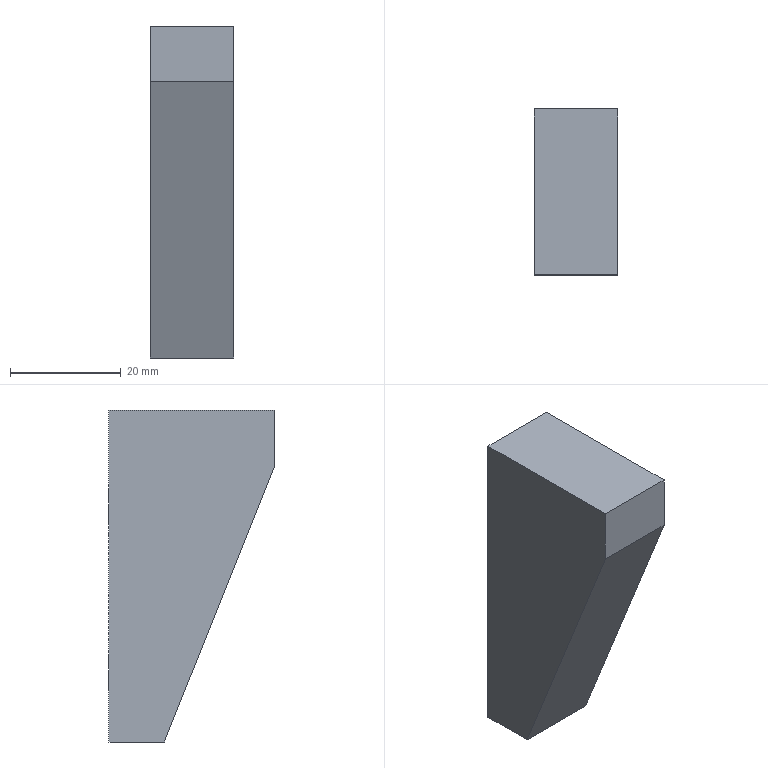Component | NX | REINFORCE_RIB_2 | 1 solid | 13 faces | box 15 x 30 x 60 mm | volume 18782 mm3 | plane 7 | cone 4 | cylinder 2 | commonest cylinder face diameters 6 x2
STEP:
#1=CARTESIAN_POINT('',(0.,0.,0.));
#2=DIRECTION('',(0.,0.,1.));
#3=DIRECTION('',(1.,0.,0.));
#4=AXIS2_PLACEMENT_3D('',#1,#2,#3);
#5=CARTESIAN_POINT('',(-1.906,179.462,226.966));
#6=VERTEX_POINT('',#5);
#7=CARTESIAN_POINT('',(-1.906,179.462,223.466));
#8=DIRECTION('',(0.,-1.,0.));
#9=DIRECTION('',(0.,0.,1.));
#10=AXIS2_PLACEMENT_3D('',#7,#8,#9);
#11=CIRCLE('',#10,3.5);
#12=CARTESIAN_POINT('',(-9.406,179.462,270.466));
#13=DIRECTION('',(0.,-1.,0.));
#14=DIRECTION('',(0.,0.,1.));
#15=AXIS2_PLACEMENT_3D('',#12,#13,#14);
#16=PLANE('',#15);
#17=CARTESIAN_POINT('',(-47.,-7.5));
#18=DIRECTION('',(1.,0.));
#19=AXIS2_PLACEMENT_2D('',#17,#18);
#20=CIRCLE('',#19,3.5);
#21=(GEOMETRIC_REPRESENTATION_CONTEXT(2)PARAMETRIC_REPRESENTATION_CONTEXT()REPRESENTATION_CONTEXT('',''));
#22=DEFINITIONAL_REPRESENTATION('',(#20),#21);
#23=PCURVE('',#16,#22);
#24=CARTESIAN_POINT('',(-1.906,179.462,223.466));
#25=DIRECTION('',(0.,1.,0.));
#26=DIRECTION('',(-1.,0.,0.));
#27=AXIS2_PLACEMENT_3D('',#24,#25,#26);
#28=CONICAL_SURFACE('',#27,3.5,0.7854);
#29=CARTESIAN_POINT('',(7.854,0.));
#30=DIRECTION('',(-1.,0.));
#31=VECTOR('',#30,1.);
#32=LINE('',#29,#31);
#33=(GEOMETRIC_REPRESENTATION_CONTEXT(2)PARAMETRIC_REPRESENTATION_CONTEXT()REPRESENTATION_CONTEXT('',''));
#34=DEFINITIONAL_REPRESENTATION('',(#32),#33);
#35=PCURVE('',#28,#34);
#36=SURFACE_CURVE('',#11,(#23,#35),.PCURVE_S1.);
#37=EDGE_CURVE('',#6,#6,#36,.T.);
#38=ORIENTED_EDGE('',*,*,#37,.T.);
#39=EDGE_LOOP('',(#38));
#40=FACE_BOUND('',#39,.T.);
#41=CARTESIAN_POINT('',(-1.906,179.462,256.966));
#42=VERTEX_POINT('',#41);
#43=CARTESIAN_POINT('',(-1.906,179.462,253.466));
#44=DIRECTION('',(0.,-1.,0.));
#45=DIRECTION('',(0.,0.,1.));
#46=AXIS2_PLACEMENT_3D('',#43,#44,#45);
#47=CIRCLE('',#46,3.5);
#48=CARTESIAN_POINT('',(-17.,-7.5));
#49=DIRECTION('',(1.,0.));
#50=AXIS2_PLACEMENT_2D('',#48,#49);
#51=CIRCLE('',#50,3.5);
#52=(GEOMETRIC_REPRESENTATION_CONTEXT(2)PARAMETRIC_REPRESENTATION_CONTEXT()REPRESENTATION_CONTEXT('',''));
#53=DEFINITIONAL_REPRESENTATION('',(#51),#52);
#54=PCURVE('',#16,#53);
#55=CARTESIAN_POINT('',(-1.906,179.462,253.466));
#56=DIRECTION('',(0.,1.,0.));
#57=DIRECTION('',(-1.,0.,0.));
#58=AXIS2_PLACEMENT_3D('',#55,#56,#57);
#59=CONICAL_SURFACE('',#58,3.5,0.7854);
#60=CARTESIAN_POINT('',(7.854,0.));
#61=DIRECTION('',(-1.,0.));
#62=VECTOR('',#61,1.);
#63=LINE('',#60,#62);
#64=(GEOMETRIC_REPRESENTATION_CONTEXT(2)PARAMETRIC_REPRESENTATION_CONTEXT()REPRESENTATION_CONTEXT('',''));
#65=DEFINITIONAL_REPRESENTATION('',(#63),#64);
#66=PCURVE('',#59,#65);
#67=SURFACE_CURVE('',#47,(#54,#66),.PCURVE_S1.);
#68=EDGE_CURVE('',#42,#42,#67,.T.);
#69=ORIENTED_EDGE('',*,*,#68,.T.);
#70=EDGE_LOOP('',(#69));
#71=FACE_BOUND('',#70,.T.);
#72=CARTESIAN_POINT('',(5.594,179.462,270.466));
#73=VERTEX_POINT('',#72);
#74=CARTESIAN_POINT('',(5.594,179.462,210.466));
#75=VERTEX_POINT('',#74);
#76=CARTESIAN_POINT('',(5.594,179.462,270.466));
#77=DIRECTION('',(0.,-0.,-1.));
#78=VECTOR('',#77,1.);
#79=LINE('',#76,#78);
#80=CARTESIAN_POINT('',(0.,-15.));
#81=DIRECTION('',(-1.,0.));
#82=VECTOR('',#81,1.);
#83=LINE('',#80,#82);
#84=(GEOMETRIC_REPRESENTATION_CONTEXT(2)PARAMETRIC_REPRESENTATION_CONTEXT()REPRESENTATION_CONTEXT('',''));
#85=DEFINITIONAL_REPRESENTATION('',(#83),#84);
#86=PCURVE('',#16,#85);
#87=CARTESIAN_POINT('',(5.594,179.462,210.466));
#88=DIRECTION('',(-1.,0.,0.));
#89=DIRECTION('',(0.,-1.,0.));
#90=AXIS2_PLACEMENT_3D('',#87,#88,#89);
#91=PLANE('',#90);
#92=CARTESIAN_POINT('',(0.,60.));
#93=DIRECTION('',(0.,-1.));
#94=VECTOR('',#93,1.);
#95=LINE('',#92,#94);
#96=(GEOMETRIC_REPRESENTATION_CONTEXT(2)PARAMETRIC_REPRESENTATION_CONTEXT()REPRESENTATION_CONTEXT('',''));
#97=DEFINITIONAL_REPRESENTATION('',(#95),#96);
#98=PCURVE('',#91,#97);
#99=SURFACE_CURVE('',#79,(#86,#98),.PCURVE_S1.);
#100=EDGE_CURVE('',#73,#75,#99,.T.);
#101=ORIENTED_EDGE('',*,*,#100,.T.);
#102=CARTESIAN_POINT('',(-9.406,179.462,210.466));
#103=VERTEX_POINT('',#102);
#104=CARTESIAN_POINT('',(-9.406,179.462,210.466));
#105=DIRECTION('',(1.,0.,0.));
#106=VECTOR('',#105,1.);
#107=LINE('',#104,#106);
#108=CARTESIAN_POINT('',(-60.,0.));
#109=DIRECTION('',(0.,-1.));
#110=VECTOR('',#109,1.);
#111=LINE('',#108,#110);
#112=(GEOMETRIC_REPRESENTATION_CONTEXT(2)PARAMETRIC_REPRESENTATION_CONTEXT()REPRESENTATION_CONTEXT('',''));
#113=DEFINITIONAL_REPRESENTATION('',(#111),#112);
#114=PCURVE('',#16,#113);
#115=CARTESIAN_POINT('',(-9.406,179.462,210.466));
#116=DIRECTION('',(0.,0.,1.));
#117=DIRECTION('',(-1.,0.,0.));
#118=AXIS2_PLACEMENT_3D('',#115,#116,#117);
#119=PLANE('',#118);
#120=CARTESIAN_POINT('',(0.,0.));
#121=DIRECTION('',(-1.,0.));
#122=VECTOR('',#121,1.);
#123=LINE('',#120,#122);
#124=(GEOMETRIC_REPRESENTATION_CONTEXT(2)PARAMETRIC_REPRESENTATION_CONTEXT()REPRESENTATION_CONTEXT('',''));
#125=DEFINITIONAL_REPRESENTATION('',(#123),#124);
#126=PCURVE('',#119,#125);
#127=SURFACE_CURVE('',#107,(#114,#126),.PCURVE_S1.);
#128=EDGE_CURVE('',#103,#75,#127,.T.);
#129=ORIENTED_EDGE('',*,*,#128,.F.);
#130=CARTESIAN_POINT('',(-9.406,179.462,270.466));
#131=VERTEX_POINT('',#130);
#132=CARTESIAN_POINT('',(-9.406,179.462,270.466));
#133=DIRECTION('',(0.,-0.,-1.));
#134=VECTOR('',#133,1.);
#135=LINE('',#132,#134);
#136=CARTESIAN_POINT('',(0.,0.));
#137=DIRECTION('',(-1.,0.));
#138=VECTOR('',#137,1.);
#139=LINE('',#136,#138);
#140=(GEOMETRIC_REPRESENTATION_CONTEXT(2)PARAMETRIC_REPRESENTATION_CONTEXT()REPRESENTATION_CONTEXT('',''));
#141=DEFINITIONAL_REPRESENTATION('',(#139),#140);
#142=PCURVE('',#16,#141);
#143=CARTESIAN_POINT('',(-9.406,179.462,210.466));
#144=DIRECTION('',(-1.,0.,0.));
#145=DIRECTION('',(0.,-1.,0.));
#146=AXIS2_PLACEMENT_3D('',#143,#144,#145);
#147=PLANE('',#146);
#148=CARTESIAN_POINT('',(0.,60.));
#149=DIRECTION('',(0.,-1.));
#150=VECTOR('',#149,1.);
#151=LINE('',#148,#150);
#152=(GEOMETRIC_REPRESENTATION_CONTEXT(2)PARAMETRIC_REPRESENTATION_CONTEXT()REPRESENTATION_CONTEXT('',''));
#153=DEFINITIONAL_REPRESENTATION('',(#151),#152);
#154=PCURVE('',#147,#153);
#155=SURFACE_CURVE('',#135,(#142,#154),.PCURVE_S1.);
#156=EDGE_CURVE('',#131,#103,#155,.T.);
#157=ORIENTED_EDGE('',*,*,#156,.F.);
#158=CARTESIAN_POINT('',(-9.406,179.462,270.466));
#159=DIRECTION('',(1.,0.,0.));
#160=VECTOR('',#159,1.);
#161=LINE('',#158,#160);
#162=CARTESIAN_POINT('',(0.,0.));
#163=DIRECTION('',(0.,-1.));
#164=VECTOR('',#163,1.);
#165=LINE('',#162,#164);
#166=(GEOMETRIC_REPRESENTATION_CONTEXT(2)PARAMETRIC_REPRESENTATION_CONTEXT()REPRESENTATION_CONTEXT('',''));
#167=DEFINITIONAL_REPRESENTATION('',(#165),#166);
#168=PCURVE('',#16,#167);
#169=CARTESIAN_POINT('',(-9.406,149.462,270.466));
#170=DIRECTION('',(0.,0.,-1.));
#171=DIRECTION('',(1.,0.,0.));
#172=AXIS2_PLACEMENT_3D('',#169,#170,#171);
#173=PLANE('',#172);
#174=CARTESIAN_POINT('',(0.,-30.));
#175=DIRECTION('',(1.,0.));
#176=VECTOR('',#175,1.);
#177=LINE('',#174,#176);
#178=(GEOMETRIC_REPRESENTATION_CONTEXT(2)PARAMETRIC_REPRESENTATION_CONTEXT()REPRESENTATION_CONTEXT('',''));
#179=DEFINITIONAL_REPRESENTATION('',(#177),#178);
#180=PCURVE('',#173,#179);
#181=SURFACE_CURVE('',#161,(#168,#180),.PCURVE_S1.);
#182=EDGE_CURVE('',#131,#73,#181,.T.);
#183=ORIENTED_EDGE('',*,*,#182,.T.);
#184=EDGE_LOOP('',(#101,#129,#157,#183));
#185=FACE_BOUND('',#184,.T.);
#186=ADVANCED_FACE('',(#40,#71,#185),#16,.F.);
#187=CARTESIAN_POINT('',(5.594,169.462,210.466));
#188=VERTEX_POINT('',#187);
#189=CARTESIAN_POINT('',(5.594,179.462,210.466));
#190=DIRECTION('',(0.,-1.,0.));
#191=VECTOR('',#190,1.);
#192=LINE('',#189,#191);
#193=CARTESIAN_POINT('',(-15.,0.));
#194=DIRECTION('',(0.,1.));
#195=VECTOR('',#194,1.);
#196=LINE('',#193,#195);
#197=(GEOMETRIC_REPRESENTATION_CONTEXT(2)PARAMETRIC_REPRESENTATION_CONTEXT()REPRESENTATION_CONTEXT('',''));
#198=DEFINITIONAL_REPRESENTATION('',(#196),#197);
#199=PCURVE('',#119,#198);
#200=CARTESIAN_POINT('',(0.,0.));
#201=DIRECTION('',(1.,0.));
#202=VECTOR('',#201,1.);
#203=LINE('',#200,#202);
#204=(GEOMETRIC_REPRESENTATION_CONTEXT(2)PARAMETRIC_REPRESENTATION_CONTEXT()REPRESENTATION_CONTEXT('',''));
#205=DEFINITIONAL_REPRESENTATION('',(#203),#204);
#206=PCURVE('',#91,#205);
#207=SURFACE_CURVE('',#192,(#199,#206),.PCURVE_S1.);
#208=EDGE_CURVE('',#75,#188,#207,.T.);
#209=ORIENTED_EDGE('',*,*,#208,.T.);
#210=CARTESIAN_POINT('',(-9.406,169.462,210.466));
#211=VERTEX_POINT('',#210);
#212=CARTESIAN_POINT('',(-9.406,169.462,210.466));
#213=DIRECTION('',(1.,0.,0.));
#214=VECTOR('',#213,1.);
#215=LINE('',#212,#214);
#216=CARTESIAN_POINT('',(0.,10.));
#217=DIRECTION('',(-1.,0.));
#218=VECTOR('',#217,1.);
#219=LINE('',#216,#218);
#220=(GEOMETRIC_REPRESENTATION_CONTEXT(2)PARAMETRIC_REPRESENTATION_CONTEXT()REPRESENTATION_CONTEXT('',''));
#221=DEFINITIONAL_REPRESENTATION('',(#219),#220);
#222=PCURVE('',#119,#221);
#223=CARTESIAN_POINT('',(-9.406,169.462,210.466));
#224=DIRECTION('',(0.,0.9285,0.3714));
#225=DIRECTION('',(0.,0.3714,-0.9285));
#226=AXIS2_PLACEMENT_3D('',#223,#224,#225);
#227=PLANE('',#226);
#228=CARTESIAN_POINT('',(0.,0.));
#229=DIRECTION('',(0.,-1.));
#230=VECTOR('',#229,1.);
#231=LINE('',#228,#230);
#232=(GEOMETRIC_REPRESENTATION_CONTEXT(2)PARAMETRIC_REPRESENTATION_CONTEXT()REPRESENTATION_CONTEXT('',''));
#233=DEFINITIONAL_REPRESENTATION('',(#231),#232);
#234=PCURVE('',#227,#233);
#235=SURFACE_CURVE('',#215,(#222,#234),.PCURVE_S1.);
#236=EDGE_CURVE('',#211,#188,#235,.T.);
#237=ORIENTED_EDGE('',*,*,#236,.F.);
#238=CARTESIAN_POINT('',(-9.406,179.462,210.466));
#239=DIRECTION('',(0.,-1.,0.));
#240=VECTOR('',#239,1.);
#241=LINE('',#238,#240);
#242=CARTESIAN_POINT('',(0.,0.));
#243=DIRECTION('',(0.,1.));
#244=VECTOR('',#243,1.);
#245=LINE('',#242,#244);
#246=(GEOMETRIC_REPRESENTATION_CONTEXT(2)PARAMETRIC_REPRESENTATION_CONTEXT()REPRESENTATION_CONTEXT('',''));
#247=DEFINITIONAL_REPRESENTATION('',(#245),#246);
#248=PCURVE('',#119,#247);
#249=CARTESIAN_POINT('',(0.,0.));
#250=DIRECTION('',(1.,0.));
#251=VECTOR('',#250,1.);
#252=LINE('',#249,#251);
#253=(GEOMETRIC_REPRESENTATION_CONTEXT(2)PARAMETRIC_REPRESENTATION_CONTEXT()REPRESENTATION_CONTEXT('',''));
#254=DEFINITIONAL_REPRESENTATION('',(#252),#253);
#255=PCURVE('',#147,#254);
#256=SURFACE_CURVE('',#241,(#248,#255),.PCURVE_S1.);
#257=EDGE_CURVE('',#103,#211,#256,.T.);
#258=ORIENTED_EDGE('',*,*,#257,.F.);
#259=ORIENTED_EDGE('',*,*,#128,.T.);
#260=EDGE_LOOP('',(#209,#237,#258,#259));
#261=FACE_BOUND('',#260,.T.);
#262=ADVANCED_FACE('',(#261),#119,.F.);
#263=CARTESIAN_POINT('',(5.594,149.462,260.466));
#264=VERTEX_POINT('',#263);
#265=CARTESIAN_POINT('',(5.594,169.462,210.466));
#266=DIRECTION('',(0.,-0.3714,0.9285));
#267=VECTOR('',#266,1.);
#268=LINE('',#265,#267);
#269=CARTESIAN_POINT('',(0.,-15.));
#270=DIRECTION('',(-1.,0.));
#271=VECTOR('',#270,1.);
#272=LINE('',#269,#271);
#273=(GEOMETRIC_REPRESENTATION_CONTEXT(2)PARAMETRIC_REPRESENTATION_CONTEXT()REPRESENTATION_CONTEXT('',''));
#274=DEFINITIONAL_REPRESENTATION('',(#272),#273);
#275=PCURVE('',#227,#274);
#276=CARTESIAN_POINT('',(10.,0.));
#277=DIRECTION('',(0.3714,0.9285));
#278=VECTOR('',#277,1.);
#279=LINE('',#276,#278);
#280=(GEOMETRIC_REPRESENTATION_CONTEXT(2)PARAMETRIC_REPRESENTATION_CONTEXT()REPRESENTATION_CONTEXT('',''));
#281=DEFINITIONAL_REPRESENTATION('',(#279),#280);
#282=PCURVE('',#91,#281);
#283=SURFACE_CURVE('',#268,(#275,#282),.PCURVE_S1.);
#284=EDGE_CURVE('',#188,#264,#283,.T.);
#285=ORIENTED_EDGE('',*,*,#284,.T.);
#286=CARTESIAN_POINT('',(-9.406,149.462,260.466));
#287=VERTEX_POINT('',#286);
#288=CARTESIAN_POINT('',(-9.406,149.462,260.466));
#289=DIRECTION('',(1.,0.,0.));
#290=VECTOR('',#289,1.);
#291=LINE('',#288,#290);
#292=CARTESIAN_POINT('',(-53.852,0.));
#293=DIRECTION('',(0.,-1.));
#294=VECTOR('',#293,1.);
#295=LINE('',#292,#294);
#296=(GEOMETRIC_REPRESENTATION_CONTEXT(2)PARAMETRIC_REPRESENTATION_CONTEXT()REPRESENTATION_CONTEXT('',''));
#297=DEFINITIONAL_REPRESENTATION('',(#295),#296);
#298=PCURVE('',#227,#297);
#299=CARTESIAN_POINT('',(-9.406,149.462,260.466));
#300=DIRECTION('',(0.,1.,0.));
#301=DIRECTION('',(-1.,0.,0.));
#302=AXIS2_PLACEMENT_3D('',#299,#300,#301);
#303=PLANE('',#302);
#304=CARTESIAN_POINT('',(0.,0.));
#305=DIRECTION('',(-1.,0.));
#306=VECTOR('',#305,1.);
#307=LINE('',#304,#306);
#308=(GEOMETRIC_REPRESENTATION_CONTEXT(2)PARAMETRIC_REPRESENTATION_CONTEXT()REPRESENTATION_CONTEXT('',''));
#309=DEFINITIONAL_REPRESENTATION('',(#307),#308);
#310=PCURVE('',#303,#309);
#311=SURFACE_CURVE('',#291,(#298,#310),.PCURVE_S1.);
#312=EDGE_CURVE('',#287,#264,#311,.T.);
#313=ORIENTED_EDGE('',*,*,#312,.F.);
#314=CARTESIAN_POINT('',(-9.406,169.462,210.466));
#315=DIRECTION('',(0.,-0.3714,0.9285));
#316=VECTOR('',#315,1.);
#317=LINE('',#314,#316);
#318=CARTESIAN_POINT('',(0.,0.));
#319=DIRECTION('',(-1.,0.));
#320=VECTOR('',#319,1.);
#321=LINE('',#318,#320);
#322=(GEOMETRIC_REPRESENTATION_CONTEXT(2)PARAMETRIC_REPRESENTATION_CONTEXT()REPRESENTATION_CONTEXT('',''));
#323=DEFINITIONAL_REPRESENTATION('',(#321),#322);
#324=PCURVE('',#227,#323);
#325=CARTESIAN_POINT('',(10.,0.));
#326=DIRECTION('',(0.3714,0.9285));
#327=VECTOR('',#326,1.);
#328=LINE('',#325,#327);
#329=(GEOMETRIC_REPRESENTATION_CONTEXT(2)PARAMETRIC_REPRESENTATION_CONTEXT()REPRESENTATION_CONTEXT('',''));
#330=DEFINITIONAL_REPRESENTATION('',(#328),#329);
#331=PCURVE('',#147,#330);
#332=SURFACE_CURVE('',#317,(#324,#331),.PCURVE_S1.);
#333=EDGE_CURVE('',#211,#287,#332,.T.);
#334=ORIENTED_EDGE('',*,*,#333,.F.);
#335=ORIENTED_EDGE('',*,*,#236,.T.);
#336=EDGE_LOOP('',(#285,#313,#334,#335));
#337=FACE_BOUND('',#336,.T.);
#338=ADVANCED_FACE('',(#337),#227,.F.);
#339=CARTESIAN_POINT('',(5.594,149.462,270.466));
#340=VERTEX_POINT('',#339);
#341=CARTESIAN_POINT('',(5.594,149.462,260.466));
#342=DIRECTION('',(0.,0.,1.));
#343=VECTOR('',#342,1.);
#344=LINE('',#341,#343);
#345=CARTESIAN_POINT('',(-15.,0.));
#346=DIRECTION('',(0.,1.));
#347=VECTOR('',#346,1.);
#348=LINE('',#345,#347);
#349=(GEOMETRIC_REPRESENTATION_CONTEXT(2)PARAMETRIC_REPRESENTATION_CONTEXT()REPRESENTATION_CONTEXT('',''));
#350=DEFINITIONAL_REPRESENTATION('',(#348),#349);
#351=PCURVE('',#303,#350);
#352=CARTESIAN_POINT('',(30.,50.));
#353=DIRECTION('',(0.,1.));
#354=VECTOR('',#353,1.);
#355=LINE('',#352,#354);
#356=(GEOMETRIC_REPRESENTATION_CONTEXT(2)PARAMETRIC_REPRESENTATION_CONTEXT()REPRESENTATION_CONTEXT('',''));
#357=DEFINITIONAL_REPRESENTATION('',(#355),#356);
#358=PCURVE('',#91,#357);
#359=SURFACE_CURVE('',#344,(#351,#358),.PCURVE_S1.);
#360=EDGE_CURVE('',#264,#340,#359,.T.);
#361=ORIENTED_EDGE('',*,*,#360,.T.);
#362=CARTESIAN_POINT('',(-9.406,149.462,270.466));
#363=VERTEX_POINT('',#362);
#364=CARTESIAN_POINT('',(-9.406,149.462,270.466));
#365=DIRECTION('',(1.,0.,0.));
#366=VECTOR('',#365,1.);
#367=LINE('',#364,#366);
#368=CARTESIAN_POINT('',(0.,10.));
#369=DIRECTION('',(-1.,0.));
#370=VECTOR('',#369,1.);
#371=LINE('',#368,#370);
#372=(GEOMETRIC_REPRESENTATION_CONTEXT(2)PARAMETRIC_REPRESENTATION_CONTEXT()REPRESENTATION_CONTEXT('',''));
#373=DEFINITIONAL_REPRESENTATION('',(#371),#372);
#374=PCURVE('',#303,#373);
#375=CARTESIAN_POINT('',(0.,0.));
#376=DIRECTION('',(1.,0.));
#377=VECTOR('',#376,1.);
#378=LINE('',#375,#377);
#379=(GEOMETRIC_REPRESENTATION_CONTEXT(2)PARAMETRIC_REPRESENTATION_CONTEXT()REPRESENTATION_CONTEXT('',''));
#380=DEFINITIONAL_REPRESENTATION('',(#378),#379);
#381=PCURVE('',#173,#380);
#382=SURFACE_CURVE('',#367,(#374,#381),.PCURVE_S1.);
#383=EDGE_CURVE('',#363,#340,#382,.T.);
#384=ORIENTED_EDGE('',*,*,#383,.F.);
#385=CARTESIAN_POINT('',(-9.406,149.462,260.466));
#386=DIRECTION('',(0.,0.,1.));
#387=VECTOR('',#386,1.);
#388=LINE('',#385,#387);
#389=CARTESIAN_POINT('',(0.,0.));
#390=DIRECTION('',(0.,1.));
#391=VECTOR('',#390,1.);
#392=LINE('',#389,#391);
#393=(GEOMETRIC_REPRESENTATION_CONTEXT(2)PARAMETRIC_REPRESENTATION_CONTEXT()REPRESENTATION_CONTEXT('',''));
#394=DEFINITIONAL_REPRESENTATION('',(#392),#393);
#395=PCURVE('',#303,#394);
#396=CARTESIAN_POINT('',(30.,50.));
#397=DIRECTION('',(0.,1.));
#398=VECTOR('',#397,1.);
#399=LINE('',#396,#398);
#400=(GEOMETRIC_REPRESENTATION_CONTEXT(2)PARAMETRIC_REPRESENTATION_CONTEXT()REPRESENTATION_CONTEXT('',''));
#401=DEFINITIONAL_REPRESENTATION('',(#399),#400);
#402=PCURVE('',#147,#401);
#403=SURFACE_CURVE('',#388,(#395,#402),.PCURVE_S1.);
#404=EDGE_CURVE('',#287,#363,#403,.T.);
#405=ORIENTED_EDGE('',*,*,#404,.F.);
#406=ORIENTED_EDGE('',*,*,#312,.T.);
#407=EDGE_LOOP('',(#361,#384,#405,#406));
#408=FACE_BOUND('',#407,.T.);
#409=ADVANCED_FACE('',(#408),#303,.F.);
#410=CARTESIAN_POINT('',(5.594,149.462,270.466));
#411=DIRECTION('',(0.,1.,0.));
#412=VECTOR('',#411,1.);
#413=LINE('',#410,#412);
#414=CARTESIAN_POINT('',(15.,0.));
#415=DIRECTION('',(0.,-1.));
#416=VECTOR('',#415,1.);
#417=LINE('',#414,#416);
#418=(GEOMETRIC_REPRESENTATION_CONTEXT(2)PARAMETRIC_REPRESENTATION_CONTEXT()REPRESENTATION_CONTEXT('',''));
#419=DEFINITIONAL_REPRESENTATION('',(#417),#418);
#420=PCURVE('',#173,#419);
#421=CARTESIAN_POINT('',(30.,60.));
#422=DIRECTION('',(-1.,0.));
#423=VECTOR('',#422,1.);
#424=LINE('',#421,#423);
#425=(GEOMETRIC_REPRESENTATION_CONTEXT(2)PARAMETRIC_REPRESENTATION_CONTEXT()REPRESENTATION_CONTEXT('',''));
#426=DEFINITIONAL_REPRESENTATION('',(#424),#425);
#427=PCURVE('',#91,#426);
#428=SURFACE_CURVE('',#413,(#420,#427),.PCURVE_S1.);
#429=EDGE_CURVE('',#340,#73,#428,.T.);
#430=ORIENTED_EDGE('',*,*,#429,.T.);
#431=ORIENTED_EDGE('',*,*,#182,.F.);
#432=CARTESIAN_POINT('',(-9.406,149.462,270.466));
#433=DIRECTION('',(0.,1.,0.));
#434=VECTOR('',#433,1.);
#435=LINE('',#432,#434);
#436=CARTESIAN_POINT('',(0.,0.));
#437=DIRECTION('',(0.,-1.));
#438=VECTOR('',#437,1.);
#439=LINE('',#436,#438);
#440=(GEOMETRIC_REPRESENTATION_CONTEXT(2)PARAMETRIC_REPRESENTATION_CONTEXT()REPRESENTATION_CONTEXT('',''));
#441=DEFINITIONAL_REPRESENTATION('',(#439),#440);
#442=PCURVE('',#173,#441);
#443=CARTESIAN_POINT('',(30.,60.));
#444=DIRECTION('',(-1.,0.));
#445=VECTOR('',#444,1.);
#446=LINE('',#443,#445);
#447=(GEOMETRIC_REPRESENTATION_CONTEXT(2)PARAMETRIC_REPRESENTATION_CONTEXT()REPRESENTATION_CONTEXT('',''));
#448=DEFINITIONAL_REPRESENTATION('',(#446),#447);
#449=PCURVE('',#147,#448);
#450=SURFACE_CURVE('',#435,(#442,#449),.PCURVE_S1.);
#451=EDGE_CURVE('',#363,#131,#450,.T.);
#452=ORIENTED_EDGE('',*,*,#451,.F.);
#453=ORIENTED_EDGE('',*,*,#383,.T.);
#454=EDGE_LOOP('',(#430,#431,#452,#453));
#455=FACE_BOUND('',#454,.T.);
#456=ADVANCED_FACE('',(#455),#173,.F.);
#457=ORIENTED_EDGE('',*,*,#156,.T.);
#458=ORIENTED_EDGE('',*,*,#257,.T.);
#459=ORIENTED_EDGE('',*,*,#333,.T.);
#460=ORIENTED_EDGE('',*,*,#404,.T.);
#461=ORIENTED_EDGE('',*,*,#451,.T.);
#462=EDGE_LOOP('',(#457,#458,#459,#460,#461));
#463=FACE_BOUND('',#462,.T.);
#464=ADVANCED_FACE('',(#463),#147,.T.);
#465=ORIENTED_EDGE('',*,*,#100,.F.);
#466=ORIENTED_EDGE('',*,*,#429,.F.);
#467=ORIENTED_EDGE('',*,*,#360,.F.);
#468=ORIENTED_EDGE('',*,*,#284,.F.);
#469=ORIENTED_EDGE('',*,*,#208,.F.);
#470=EDGE_LOOP('',(#465,#466,#467,#468,#469));
#471=FACE_BOUND('',#470,.T.);
#472=ADVANCED_FACE('',(#471),#91,.F.);
#473=CARTESIAN_POINT('',(-1.906,167.462,250.466));
#474=VERTEX_POINT('',#473);
#475=CARTESIAN_POINT('',(-1.906,167.462,256.466));
#476=VERTEX_POINT('',#475);
#477=CARTESIAN_POINT('',(-1.906,167.462,253.466));
#478=DIRECTION('',(0.,1.,-0.));
#479=DIRECTION('',(0.,0.,1.));
#480=AXIS2_PLACEMENT_3D('',#477,#478,#479);
#481=CIRCLE('',#480,3.);
#482=CARTESIAN_POINT('',(-1.906,167.462,253.466));
#483=DIRECTION('',(0.,1.,-0.));
#484=DIRECTION('',(0.,-0.,-1.));
#485=AXIS2_PLACEMENT_3D('',#482,#483,#484);
#486=CONICAL_SURFACE('',#485,3.,1.03);
#487=CARTESIAN_POINT('',(-3.142,0.));
#488=DIRECTION('',(1.,0.));
#489=VECTOR('',#488,1.);
#490=LINE('',#487,#489);
#491=(GEOMETRIC_REPRESENTATION_CONTEXT(2)PARAMETRIC_REPRESENTATION_CONTEXT()REPRESENTATION_CONTEXT('',''));
#492=DEFINITIONAL_REPRESENTATION('',(#490),#491);
#493=PCURVE('',#486,#492);
#494=CARTESIAN_POINT('',(-1.906,179.462,253.466));
#495=DIRECTION('',(0.,-1.,0.));
#496=DIRECTION('',(0.,0.,1.));
#497=AXIS2_PLACEMENT_3D('',#494,#495,#496);
#498=CYLINDRICAL_SURFACE('',#497,3.);
#499=CARTESIAN_POINT('',(6.283,12.));
#500=DIRECTION('',(-1.,0.));
#501=VECTOR('',#500,1.);
#502=LINE('',#499,#501);
#503=(GEOMETRIC_REPRESENTATION_CONTEXT(2)PARAMETRIC_REPRESENTATION_CONTEXT()REPRESENTATION_CONTEXT('',''));
#504=DEFINITIONAL_REPRESENTATION('',(#502),#503);
#505=PCURVE('',#498,#504);
#506=SURFACE_CURVE('',#481,(#493,#505),.PCURVE_S1.);
#507=EDGE_CURVE('',#474,#476,#506,.T.);
#508=ORIENTED_EDGE('',*,*,#507,.F.);
#509=CARTESIAN_POINT('',(-1.906,165.659,253.466));
#510=VERTEX_POINT('',#509);
#511=CARTESIAN_POINT('',(-1.906,165.659,253.466));
#512=CARTESIAN_POINT('',(-1.906,167.462,250.466));
#513=B_SPLINE_CURVE_WITH_KNOTS('',1,(#511,#512),.UNSPECIFIED.,.F.,.F.,(2,2),(-3.5,0.),.PIECEWISE_BEZIER_KNOTS.);
#514=CARTESIAN_POINT('',(0.,0.));
#515=DIRECTION('',(0.,1.));
#516=VECTOR('',#515,1.);
#517=LINE('',#514,#516);
#518=(GEOMETRIC_REPRESENTATION_CONTEXT(2)PARAMETRIC_REPRESENTATION_CONTEXT()REPRESENTATION_CONTEXT('',''));
#519=DEFINITIONAL_REPRESENTATION('',(#517),#518);
#520=PCURVE('',#486,#519);
#521=CARTESIAN_POINT('',(6.283,0.));
#522=DIRECTION('',(0.,1.));
#523=VECTOR('',#522,1.);
#524=LINE('',#521,#523);
#525=(GEOMETRIC_REPRESENTATION_CONTEXT(2)PARAMETRIC_REPRESENTATION_CONTEXT()REPRESENTATION_CONTEXT('',''));
#526=DEFINITIONAL_REPRESENTATION('',(#524),#525);
#527=PCURVE('',#486,#526);
#528=SEAM_CURVE('',#513,(#520,#527),.PCURVE_S1.);
#529=EDGE_CURVE('',#510,#474,#528,.T.);
#530=ORIENTED_EDGE('',*,*,#529,.F.);
#531=ORIENTED_EDGE('',*,*,#529,.T.);
#532=CARTESIAN_POINT('',(-1.906,167.462,253.466));
#533=DIRECTION('',(0.,1.,-0.));
#534=DIRECTION('',(0.,0.,1.));
#535=AXIS2_PLACEMENT_3D('',#532,#533,#534);
#536=CIRCLE('',#535,3.);
#537=CARTESIAN_POINT('',(3.142,0.));
#538=DIRECTION('',(1.,0.));
#539=VECTOR('',#538,1.);
#540=LINE('',#537,#539);
#541=(GEOMETRIC_REPRESENTATION_CONTEXT(2)PARAMETRIC_REPRESENTATION_CONTEXT()REPRESENTATION_CONTEXT('',''));
#542=DEFINITIONAL_REPRESENTATION('',(#540),#541);
#543=PCURVE('',#486,#542);
#544=CARTESIAN_POINT('',(6.283,12.));
#545=DIRECTION('',(-1.,0.));
#546=VECTOR('',#545,1.);
#547=LINE('',#544,#546);
#548=(GEOMETRIC_REPRESENTATION_CONTEXT(2)PARAMETRIC_REPRESENTATION_CONTEXT()REPRESENTATION_CONTEXT('',''));
#549=DEFINITIONAL_REPRESENTATION('',(#547),#548);
#550=PCURVE('',#498,#549);
#551=SURFACE_CURVE('',#536,(#543,#550),.PCURVE_S1.);
#552=EDGE_CURVE('',#476,#474,#551,.T.);
#553=ORIENTED_EDGE('',*,*,#552,.F.);
#554=EDGE_LOOP('',(#508,#530,#531,#553));
#555=FACE_BOUND('',#554,.F.);
#556=ADVANCED_FACE('',(#555),#486,.F.);
#557=CARTESIAN_POINT('',(-1.906,178.962,256.466));
#558=VERTEX_POINT('',#557);
#559=CARTESIAN_POINT('',(1.094,178.962,253.466));
#560=VERTEX_POINT('',#559);
#561=CARTESIAN_POINT('',(-1.906,178.962,253.466));
#562=DIRECTION('',(0.,1.,0.));
#563=DIRECTION('',(1.,0.,0.));
#564=AXIS2_PLACEMENT_3D('',#561,#562,#563);
#565=CIRCLE('',#564,3.);
#566=CARTESIAN_POINT('',(10.996,0.5));
#567=DIRECTION('',(-1.,0.));
#568=VECTOR('',#567,1.);
#569=LINE('',#566,#568);
#570=(GEOMETRIC_REPRESENTATION_CONTEXT(2)PARAMETRIC_REPRESENTATION_CONTEXT()REPRESENTATION_CONTEXT('',''));
#571=DEFINITIONAL_REPRESENTATION('',(#569),#570);
#572=PCURVE('',#498,#571);
#573=CARTESIAN_POINT('',(-3.142,-0.5));
#574=DIRECTION('',(1.,0.));
#575=VECTOR('',#574,1.);
#576=LINE('',#573,#575);
#577=(GEOMETRIC_REPRESENTATION_CONTEXT(2)PARAMETRIC_REPRESENTATION_CONTEXT()REPRESENTATION_CONTEXT('',''));
#578=DEFINITIONAL_REPRESENTATION('',(#576),#577);
#579=PCURVE('',#59,#578);
#580=SURFACE_CURVE('',#565,(#572,#579),.PCURVE_S1.);
#581=EDGE_CURVE('',#558,#560,#580,.T.);
#582=ORIENTED_EDGE('',*,*,#581,.F.);
#583=CARTESIAN_POINT('',(-1.906,178.962,256.466));
#584=CARTESIAN_POINT('',(-1.906,167.462,256.466));
#585=B_SPLINE_CURVE_WITH_KNOTS('',1,(#583,#584),.UNSPECIFIED.,.F.,.F.,(2,2),(0.5,12.),.PIECEWISE_BEZIER_KNOTS.);
#586=CARTESIAN_POINT('',(6.283,0.));
#587=DIRECTION('',(0.,1.));
#588=VECTOR('',#587,1.);
#589=LINE('',#586,#588);
#590=(GEOMETRIC_REPRESENTATION_CONTEXT(2)PARAMETRIC_REPRESENTATION_CONTEXT()REPRESENTATION_CONTEXT('',''));
#591=DEFINITIONAL_REPRESENTATION('',(#589),#590);
#592=PCURVE('',#498,#591);
#593=CARTESIAN_POINT('',(0.,0.));
#594=DIRECTION('',(0.,1.));
#595=VECTOR('',#594,1.);
#596=LINE('',#593,#595);
#597=(GEOMETRIC_REPRESENTATION_CONTEXT(2)PARAMETRIC_REPRESENTATION_CONTEXT()REPRESENTATION_CONTEXT('',''));
#598=DEFINITIONAL_REPRESENTATION('',(#596),#597);
#599=PCURVE('',#498,#598);
#600=SEAM_CURVE('',#585,(#592,#599),.PCURVE_S1.);
#601=EDGE_CURVE('',#558,#476,#600,.T.);
#602=ORIENTED_EDGE('',*,*,#601,.T.);
#603=ORIENTED_EDGE('',*,*,#552,.T.);
#604=ORIENTED_EDGE('',*,*,#507,.T.);
#605=ORIENTED_EDGE('',*,*,#601,.F.);
#606=CARTESIAN_POINT('',(-1.906,178.962,253.466));
#607=DIRECTION('',(0.,1.,0.));
#608=DIRECTION('',(1.,0.,0.));
#609=AXIS2_PLACEMENT_3D('',#606,#607,#608);
#610=CIRCLE('',#609,3.);
#611=CARTESIAN_POINT('',(4.712,0.5));
#612=DIRECTION('',(-1.,0.));
#613=VECTOR('',#612,1.);
#614=LINE('',#611,#613);
#615=(GEOMETRIC_REPRESENTATION_CONTEXT(2)PARAMETRIC_REPRESENTATION_CONTEXT()REPRESENTATION_CONTEXT('',''));
#616=DEFINITIONAL_REPRESENTATION('',(#614),#615);
#617=PCURVE('',#498,#616);
#618=CARTESIAN_POINT('',(3.142,-0.5));
#619=DIRECTION('',(1.,0.));
#620=VECTOR('',#619,1.);
#621=LINE('',#618,#620);
#622=(GEOMETRIC_REPRESENTATION_CONTEXT(2)PARAMETRIC_REPRESENTATION_CONTEXT()REPRESENTATION_CONTEXT('',''));
#623=DEFINITIONAL_REPRESENTATION('',(#621),#622);
#624=PCURVE('',#59,#623);
#625=SURFACE_CURVE('',#610,(#617,#624),.PCURVE_S1.);
#626=EDGE_CURVE('',#560,#558,#625,.T.);
#627=ORIENTED_EDGE('',*,*,#626,.F.);
#628=EDGE_LOOP('',(#582,#602,#603,#604,#605,#627));
#629=FACE_BOUND('',#628,.F.);
#630=ADVANCED_FACE('',(#629),#498,.F.);
#631=ORIENTED_EDGE('',*,*,#581,.T.);
#632=ORIENTED_EDGE('',*,*,#626,.T.);
#633=CARTESIAN_POINT('',(-1.906,178.962,256.466));
#634=CARTESIAN_POINT('',(-1.906,179.462,256.966));
#635=B_SPLINE_CURVE_WITH_KNOTS('',1,(#633,#634),.UNSPECIFIED.,.F.,.F.,(2,2),(-0.7071,0.),.PIECEWISE_BEZIER_KNOTS.);
#636=CARTESIAN_POINT('',(7.854,0.));
#637=DIRECTION('',(0.,1.));
#638=VECTOR('',#637,1.);
#639=LINE('',#636,#638);
#640=(GEOMETRIC_REPRESENTATION_CONTEXT(2)PARAMETRIC_REPRESENTATION_CONTEXT()REPRESENTATION_CONTEXT('',''));
#641=DEFINITIONAL_REPRESENTATION('',(#639),#640);
#642=PCURVE('',#59,#641);
#643=CARTESIAN_POINT('',(1.571,0.));
#644=DIRECTION('',(0.,1.));
#645=VECTOR('',#644,1.);
#646=LINE('',#643,#645);
#647=(GEOMETRIC_REPRESENTATION_CONTEXT(2)PARAMETRIC_REPRESENTATION_CONTEXT()REPRESENTATION_CONTEXT('',''));
#648=DEFINITIONAL_REPRESENTATION('',(#646),#647);
#649=PCURVE('',#59,#648);
#650=SEAM_CURVE('',#635,(#642,#649),.PCURVE_S1.);
#651=EDGE_CURVE('',#558,#42,#650,.T.);
#652=ORIENTED_EDGE('',*,*,#651,.T.);
#653=ORIENTED_EDGE('',*,*,#68,.T.);
#654=ORIENTED_EDGE('',*,*,#651,.F.);
#655=EDGE_LOOP('',(#631,#632,#652,#653,#654));
#656=FACE_BOUND('',#655,.F.);
#657=ADVANCED_FACE('',(#656),#59,.F.);
#658=CARTESIAN_POINT('',(-1.906,167.462,220.466));
#659=VERTEX_POINT('',#658);
#660=CARTESIAN_POINT('',(-1.906,167.462,226.466));
#661=VERTEX_POINT('',#660);
#662=CARTESIAN_POINT('',(-1.906,167.462,223.466));
#663=DIRECTION('',(0.,1.,-0.));
#664=DIRECTION('',(0.,0.,1.));
#665=AXIS2_PLACEMENT_3D('',#662,#663,#664);
#666=CIRCLE('',#665,3.);
#667=CARTESIAN_POINT('',(-1.906,167.462,223.466));
#668=DIRECTION('',(0.,1.,-0.));
#669=DIRECTION('',(0.,-0.,-1.));
#670=AXIS2_PLACEMENT_3D('',#667,#668,#669);
#671=CONICAL_SURFACE('',#670,3.,1.03);
#672=CARTESIAN_POINT('',(-3.142,0.));
#673=DIRECTION('',(1.,0.));
#674=VECTOR('',#673,1.);
#675=LINE('',#672,#674);
#676=(GEOMETRIC_REPRESENTATION_CONTEXT(2)PARAMETRIC_REPRESENTATION_CONTEXT()REPRESENTATION_CONTEXT('',''));
#677=DEFINITIONAL_REPRESENTATION('',(#675),#676);
#678=PCURVE('',#671,#677);
#679=CARTESIAN_POINT('',(-1.906,179.462,223.466));
#680=DIRECTION('',(0.,-1.,0.));
#681=DIRECTION('',(0.,0.,1.));
#682=AXIS2_PLACEMENT_3D('',#679,#680,#681);
#683=CYLINDRICAL_SURFACE('',#682,3.);
#684=CARTESIAN_POINT('',(6.283,12.));
#685=DIRECTION('',(-1.,0.));
#686=VECTOR('',#685,1.);
#687=LINE('',#684,#686);
#688=(GEOMETRIC_REPRESENTATION_CONTEXT(2)PARAMETRIC_REPRESENTATION_CONTEXT()REPRESENTATION_CONTEXT('',''));
#689=DEFINITIONAL_REPRESENTATION('',(#687),#688);
#690=PCURVE('',#683,#689);
#691=SURFACE_CURVE('',#666,(#678,#690),.PCURVE_S1.);
#692=EDGE_CURVE('',#659,#661,#691,.T.);
#693=ORIENTED_EDGE('',*,*,#692,.F.);
#694=CARTESIAN_POINT('',(-1.906,165.659,223.466));
#695=VERTEX_POINT('',#694);
#696=CARTESIAN_POINT('',(-1.906,165.659,223.466));
#697=CARTESIAN_POINT('',(-1.906,167.462,220.466));
#698=B_SPLINE_CURVE_WITH_KNOTS('',1,(#696,#697),.UNSPECIFIED.,.F.,.F.,(2,2),(-3.5,0.),.PIECEWISE_BEZIER_KNOTS.);
#699=CARTESIAN_POINT('',(0.,0.));
#700=DIRECTION('',(0.,1.));
#701=VECTOR('',#700,1.);
#702=LINE('',#699,#701);
#703=(GEOMETRIC_REPRESENTATION_CONTEXT(2)PARAMETRIC_REPRESENTATION_CONTEXT()REPRESENTATION_CONTEXT('',''));
#704=DEFINITIONAL_REPRESENTATION('',(#702),#703);
#705=PCURVE('',#671,#704);
#706=CARTESIAN_POINT('',(6.283,0.));
#707=DIRECTION('',(0.,1.));
#708=VECTOR('',#707,1.);
#709=LINE('',#706,#708);
#710=(GEOMETRIC_REPRESENTATION_CONTEXT(2)PARAMETRIC_REPRESENTATION_CONTEXT()REPRESENTATION_CONTEXT('',''));
#711=DEFINITIONAL_REPRESENTATION('',(#709),#710);
#712=PCURVE('',#671,#711);
#713=SEAM_CURVE('',#698,(#705,#712),.PCURVE_S1.);
#714=EDGE_CURVE('',#695,#659,#713,.T.);
#715=ORIENTED_EDGE('',*,*,#714,.F.);
#716=ORIENTED_EDGE('',*,*,#714,.T.);
#717=CARTESIAN_POINT('',(-1.906,167.462,223.466));
#718=DIRECTION('',(0.,1.,-0.));
#719=DIRECTION('',(0.,0.,1.));
#720=AXIS2_PLACEMENT_3D('',#717,#718,#719);
#721=CIRCLE('',#720,3.);
#722=CARTESIAN_POINT('',(3.142,0.));
#723=DIRECTION('',(1.,0.));
#724=VECTOR('',#723,1.);
#725=LINE('',#722,#724);
#726=(GEOMETRIC_REPRESENTATION_CONTEXT(2)PARAMETRIC_REPRESENTATION_CONTEXT()REPRESENTATION_CONTEXT('',''));
#727=DEFINITIONAL_REPRESENTATION('',(#725),#726);
#728=PCURVE('',#671,#727);
#729=CARTESIAN_POINT('',(6.283,12.));
#730=DIRECTION('',(-1.,0.));
#731=VECTOR('',#730,1.);
#732=LINE('',#729,#731);
#733=(GEOMETRIC_REPRESENTATION_CONTEXT(2)PARAMETRIC_REPRESENTATION_CONTEXT()REPRESENTATION_CONTEXT('',''));
#734=DEFINITIONAL_REPRESENTATION('',(#732),#733);
#735=PCURVE('',#683,#734);
#736=SURFACE_CURVE('',#721,(#728,#735),.PCURVE_S1.);
#737=EDGE_CURVE('',#661,#659,#736,.T.);
#738=ORIENTED_EDGE('',*,*,#737,.F.);
#739=EDGE_LOOP('',(#693,#715,#716,#738));
#740=FACE_BOUND('',#739,.F.);
#741=ADVANCED_FACE('',(#740),#671,.F.);
#742=CARTESIAN_POINT('',(-1.906,178.962,226.466));
#743=VERTEX_POINT('',#742);
#744=CARTESIAN_POINT('',(1.094,178.962,223.466));
#745=VERTEX_POINT('',#744);
#746=CARTESIAN_POINT('',(-1.906,178.962,223.466));
#747=DIRECTION('',(0.,1.,0.));
#748=DIRECTION('',(1.,0.,0.));
#749=AXIS2_PLACEMENT_3D('',#746,#747,#748);
#750=CIRCLE('',#749,3.);
#751=CARTESIAN_POINT('',(10.996,0.5));
#752=DIRECTION('',(-1.,0.));
#753=VECTOR('',#752,1.);
#754=LINE('',#751,#753);
#755=(GEOMETRIC_REPRESENTATION_CONTEXT(2)PARAMETRIC_REPRESENTATION_CONTEXT()REPRESENTATION_CONTEXT('',''));
#756=DEFINITIONAL_REPRESENTATION('',(#754),#755);
#757=PCURVE('',#683,#756);
#758=CARTESIAN_POINT('',(-3.142,-0.5));
#759=DIRECTION('',(1.,0.));
#760=VECTOR('',#759,1.);
#761=LINE('',#758,#760);
#762=(GEOMETRIC_REPRESENTATION_CONTEXT(2)PARAMETRIC_REPRESENTATION_CONTEXT()REPRESENTATION_CONTEXT('',''));
#763=DEFINITIONAL_REPRESENTATION('',(#761),#762);
#764=PCURVE('',#28,#763);
#765=SURFACE_CURVE('',#750,(#757,#764),.PCURVE_S1.);
#766=EDGE_CURVE('',#743,#745,#765,.T.);
#767=ORIENTED_EDGE('',*,*,#766,.F.);
#768=CARTESIAN_POINT('',(-1.906,178.962,226.466));
#769=CARTESIAN_POINT('',(-1.906,167.462,226.466));
#770=B_SPLINE_CURVE_WITH_KNOTS('',1,(#768,#769),.UNSPECIFIED.,.F.,.F.,(2,2),(0.5,12.),.PIECEWISE_BEZIER_KNOTS.);
#771=CARTESIAN_POINT('',(6.283,0.));
#772=DIRECTION('',(0.,1.));
#773=VECTOR('',#772,1.);
#774=LINE('',#771,#773);
#775=(GEOMETRIC_REPRESENTATION_CONTEXT(2)PARAMETRIC_REPRESENTATION_CONTEXT()REPRESENTATION_CONTEXT('',''));
#776=DEFINITIONAL_REPRESENTATION('',(#774),#775);
#777=PCURVE('',#683,#776);
#778=CARTESIAN_POINT('',(0.,0.));
#779=DIRECTION('',(0.,1.));
#780=VECTOR('',#779,1.);
#781=LINE('',#778,#780);
#782=(GEOMETRIC_REPRESENTATION_CONTEXT(2)PARAMETRIC_REPRESENTATION_CONTEXT()REPRESENTATION_CONTEXT('',''));
#783=DEFINITIONAL_REPRESENTATION('',(#781),#782);
#784=PCURVE('',#683,#783);
#785=SEAM_CURVE('',#770,(#777,#784),.PCURVE_S1.);
#786=EDGE_CURVE('',#743,#661,#785,.T.);
#787=ORIENTED_EDGE('',*,*,#786,.T.);
#788=ORIENTED_EDGE('',*,*,#737,.T.);
#789=ORIENTED_EDGE('',*,*,#692,.T.);
#790=ORIENTED_EDGE('',*,*,#786,.F.);
#791=CARTESIAN_POINT('',(-1.906,178.962,223.466));
#792=DIRECTION('',(0.,1.,0.));
#793=DIRECTION('',(1.,0.,0.));
#794=AXIS2_PLACEMENT_3D('',#791,#792,#793);
#795=CIRCLE('',#794,3.);
#796=CARTESIAN_POINT('',(4.712,0.5));
#797=DIRECTION('',(-1.,0.));
#798=VECTOR('',#797,1.);
#799=LINE('',#796,#798);
#800=(GEOMETRIC_REPRESENTATION_CONTEXT(2)PARAMETRIC_REPRESENTATION_CONTEXT()REPRESENTATION_CONTEXT('',''));
#801=DEFINITIONAL_REPRESENTATION('',(#799),#800);
#802=PCURVE('',#683,#801);
#803=CARTESIAN_POINT('',(3.142,-0.5));
#804=DIRECTION('',(1.,0.));
#805=VECTOR('',#804,1.);
#806=LINE('',#803,#805);
#807=(GEOMETRIC_REPRESENTATION_CONTEXT(2)PARAMETRIC_REPRESENTATION_CONTEXT()REPRESENTATION_CONTEXT('',''));
#808=DEFINITIONAL_REPRESENTATION('',(#806),#807);
#809=PCURVE('',#28,#808);
#810=SURFACE_CURVE('',#795,(#802,#809),.PCURVE_S1.);
#811=EDGE_CURVE('',#745,#743,#810,.T.);
#812=ORIENTED_EDGE('',*,*,#811,.F.);
#813=EDGE_LOOP('',(#767,#787,#788,#789,#790,#812));
#814=FACE_BOUND('',#813,.F.);
#815=ADVANCED_FACE('',(#814),#683,.F.);
#816=ORIENTED_EDGE('',*,*,#766,.T.);
#817=ORIENTED_EDGE('',*,*,#811,.T.);
#818=CARTESIAN_POINT('',(-1.906,178.962,226.466));
#819=CARTESIAN_POINT('',(-1.906,179.462,226.966));
#820=B_SPLINE_CURVE_WITH_KNOTS('',1,(#818,#819),.UNSPECIFIED.,.F.,.F.,(2,2),(-0.7071,0.),.PIECEWISE_BEZIER_KNOTS.);
#821=CARTESIAN_POINT('',(7.854,0.));
#822=DIRECTION('',(0.,1.));
#823=VECTOR('',#822,1.);
#824=LINE('',#821,#823);
#825=(GEOMETRIC_REPRESENTATION_CONTEXT(2)PARAMETRIC_REPRESENTATION_CONTEXT()REPRESENTATION_CONTEXT('',''));
#826=DEFINITIONAL_REPRESENTATION('',(#824),#825);
#827=PCURVE('',#28,#826);
#828=CARTESIAN_POINT('',(1.571,0.));
#829=DIRECTION('',(0.,1.));
#830=VECTOR('',#829,1.);
#831=LINE('',#828,#830);
#832=(GEOMETRIC_REPRESENTATION_CONTEXT(2)PARAMETRIC_REPRESENTATION_CONTEXT()REPRESENTATION_CONTEXT('',''));
#833=DEFINITIONAL_REPRESENTATION('',(#831),#832);
#834=PCURVE('',#28,#833);
#835=SEAM_CURVE('',#820,(#827,#834),.PCURVE_S1.);
#836=EDGE_CURVE('',#743,#6,#835,.T.);
#837=ORIENTED_EDGE('',*,*,#836,.T.);
#838=ORIENTED_EDGE('',*,*,#37,.T.);
#839=ORIENTED_EDGE('',*,*,#836,.F.);
#840=EDGE_LOOP('',(#816,#817,#837,#838,#839));
#841=FACE_BOUND('',#840,.F.);
#842=ADVANCED_FACE('',(#841),#28,.F.);
#843=CLOSED_SHELL('',(#186,#262,#338,#409,#456,#464,#472,#556,#630,#657,#741,#815,#842));
#844=MANIFOLD_SOLID_BREP('',#843);
#845=(LENGTH_UNIT()NAMED_UNIT(*)SI_UNIT(.MILLI.,.METRE.));
#846=UNCERTAINTY_MEASURE_WITH_UNIT(LENGTH_MEASURE(0.000005),#845,'','');
#847=(NAMED_UNIT(*)PLANE_ANGLE_UNIT()SI_UNIT($,.RADIAN.));
#848=(NAMED_UNIT(*)SI_UNIT($,.STERADIAN.)SOLID_ANGLE_UNIT());
#849=(GEOMETRIC_REPRESENTATION_CONTEXT(3)GLOBAL_UNCERTAINTY_ASSIGNED_CONTEXT((#846))GLOBAL_UNIT_ASSIGNED_CONTEXT((#845,#847,#848))REPRESENTATION_CONTEXT('',''));
#850=ADVANCED_BREP_SHAPE_REPRESENTATION('',(#4,#844),#849);